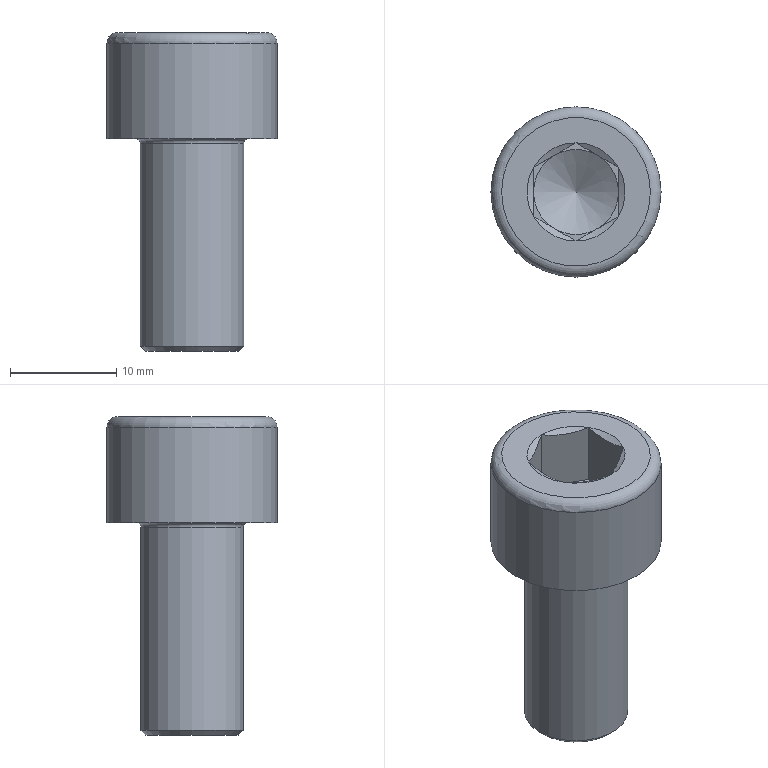Component | NX | GB-T70_1-2000_M10X20 | 1 solid | 27 faces | volume 3113 mm3 | plane 15 | cone 8 | cylinder 2 | torus 2 | commonest cylinder face diameters 9.732 x1 16 x1